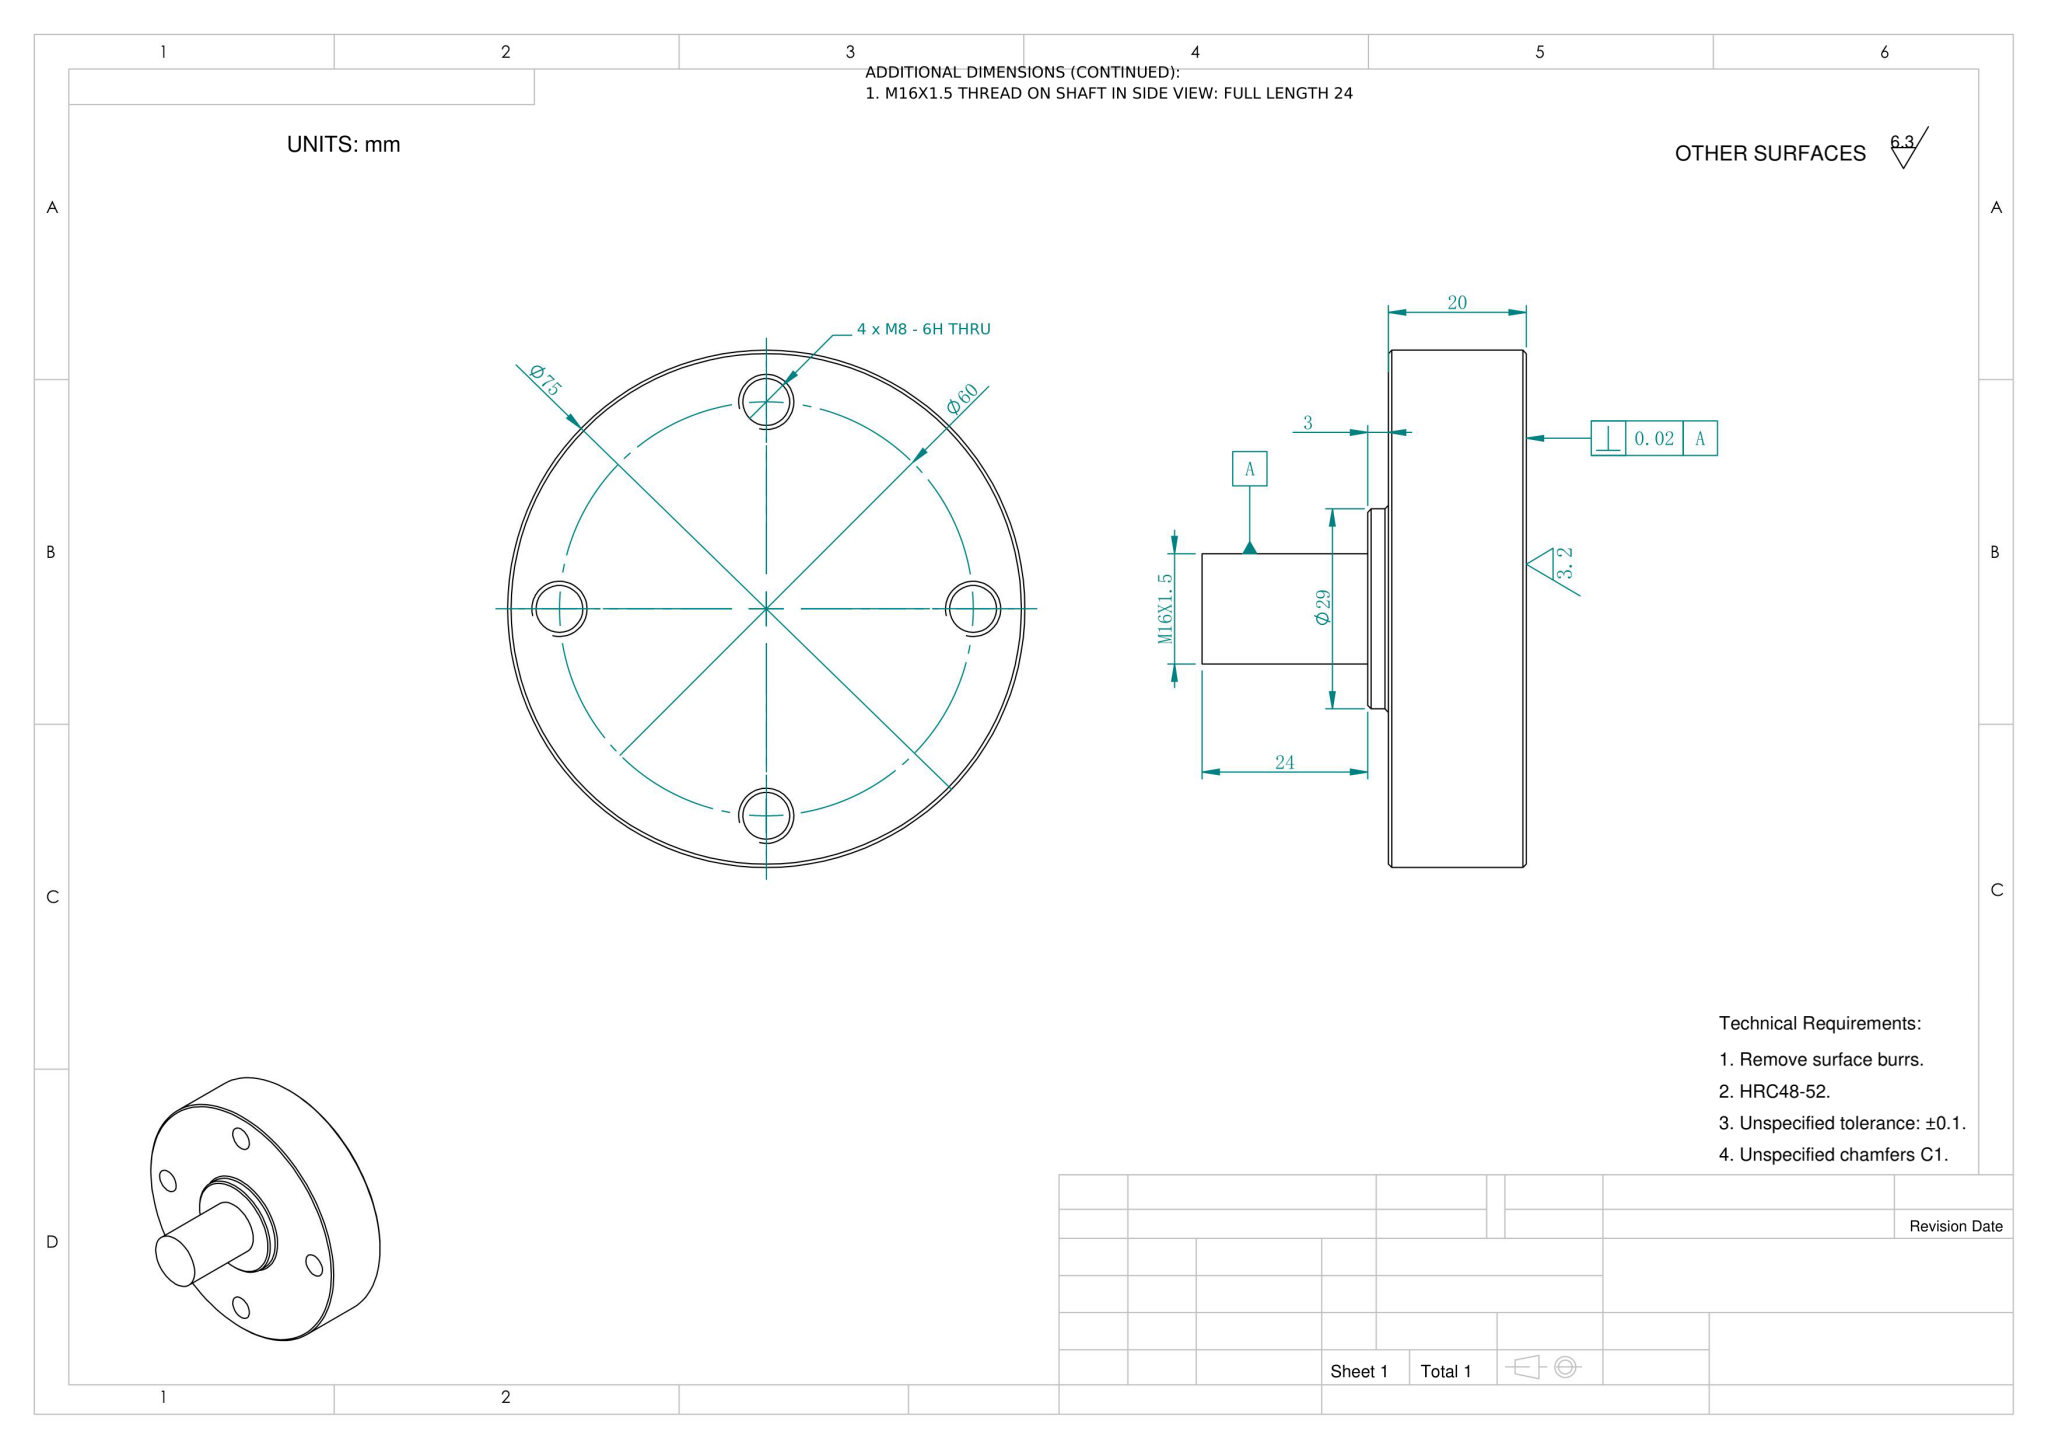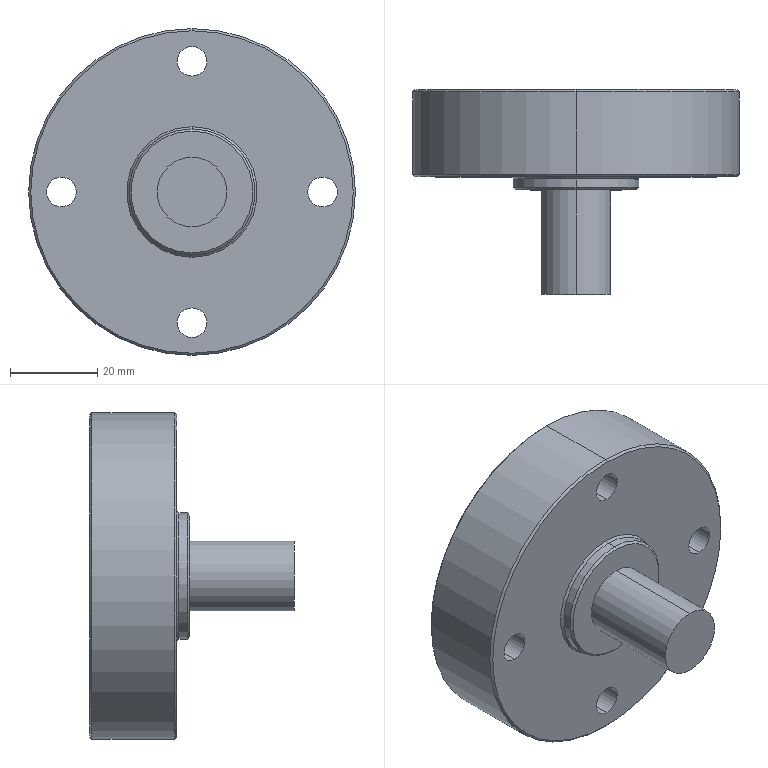Part | NX | mm | 1 solid | 26 faces | box 75 x 47 x 75 mm | volume 92201 mm3 | cylinder 14 | cone 8 | plane 4 | commonest cylinder face diameters 6.8 x8 75 x2 29 x2 16 x2
STEP:
#1=COLOUR_RGB('',0.7922,0.8196,0.9333);
#2=FILL_AREA_STYLE_COLOUR('',#1);
#3=FILL_AREA_STYLE('',(#2));
#4=SURFACE_STYLE_FILL_AREA(#3);
#5=SURFACE_SIDE_STYLE('',(#4));
#6=SURFACE_STYLE_USAGE(.BOTH.,#5);
#7=PRESENTATION_STYLE_ASSIGNMENT((#6));
#8=CARTESIAN_POINT('',(0.,27.,-37.));
#9=VERTEX_POINT('',#8);
#10=CARTESIAN_POINT('',(0.,27.,37.));
#11=VERTEX_POINT('',#10);
#12=CARTESIAN_POINT('',(0.,27.,0.));
#13=DIRECTION('',(0.,-1.,0.));
#14=DIRECTION('',(0.,0.,-1.));
#15=AXIS2_PLACEMENT_3D('',#12,#13,#14);
#16=CIRCLE('',#15,37.);
#17=EDGE_CURVE('',#9,#11,#16,.T.);
#18=ORIENTED_EDGE('',*,*,#17,.F.);
#19=CARTESIAN_POINT('',(0.,27.5,-37.5));
#20=VERTEX_POINT('',#19);
#21=CARTESIAN_POINT('',(0.,27.5,-37.5));
#22=DIRECTION('',(0.,0.7071,-0.7071));
#23=VECTOR('',#22,1000.);
#24=LINE('',#21,#23);
#25=EDGE_CURVE('',#9,#20,#24,.T.);
#26=ORIENTED_EDGE('',*,*,#25,.T.);
#27=CARTESIAN_POINT('',(0.,27.5,37.5));
#28=VERTEX_POINT('',#27);
#29=CARTESIAN_POINT('',(0.,27.5,0.));
#30=DIRECTION('',(0.,1.,0.));
#31=DIRECTION('',(0.,0.,-1.));
#32=AXIS2_PLACEMENT_3D('',#29,#30,#31);
#33=CIRCLE('',#32,37.5);
#34=EDGE_CURVE('',#28,#20,#33,.T.);
#35=ORIENTED_EDGE('',*,*,#34,.F.);
#36=CARTESIAN_POINT('',(0.,27.5,37.5));
#37=DIRECTION('',(0.,0.7071,0.7071));
#38=VECTOR('',#37,1000.);
#39=LINE('',#36,#38);
#40=EDGE_CURVE('',#11,#28,#39,.T.);
#41=ORIENTED_EDGE('',*,*,#40,.F.);
#42=EDGE_LOOP('',(#18,#26,#35,#41));
#43=FACE_OUTER_BOUND('',#42,.T.);
#44=CARTESIAN_POINT('',(0.,27.5,0.));
#45=DIRECTION('',(0.,1.,0.));
#46=DIRECTION('',(0.,0.,1.));
#47=AXIS2_PLACEMENT_3D('',#44,#45,#46);
#48=CONICAL_SURFACE('',#47,37.5,0.7854);
#49=ADVANCED_FACE('',(#43),#48,.T.);
#50=CARTESIAN_POINT('',(0.,47.,37.));
#51=VERTEX_POINT('',#50);
#52=CARTESIAN_POINT('',(0.,47.,-37.));
#53=VERTEX_POINT('',#52);
#54=CARTESIAN_POINT('',(0.,47.,0.));
#55=DIRECTION('',(0.,1.,0.));
#56=DIRECTION('',(0.,0.,1.));
#57=AXIS2_PLACEMENT_3D('',#54,#55,#56);
#58=CIRCLE('',#57,37.);
#59=EDGE_CURVE('',#51,#53,#58,.T.);
#60=ORIENTED_EDGE('',*,*,#59,.F.);
#61=CARTESIAN_POINT('',(0.,46.5,37.5));
#62=VERTEX_POINT('',#61);
#63=CARTESIAN_POINT('',(0.,47.,37.));
#64=DIRECTION('',(0.,-0.7071,0.7071));
#65=VECTOR('',#64,1000.);
#66=LINE('',#63,#65);
#67=EDGE_CURVE('',#51,#62,#66,.T.);
#68=ORIENTED_EDGE('',*,*,#67,.T.);
#69=CARTESIAN_POINT('',(0.,46.5,-37.5));
#70=VERTEX_POINT('',#69);
#71=CARTESIAN_POINT('',(0.,46.5,0.));
#72=DIRECTION('',(0.,-1.,0.));
#73=DIRECTION('',(0.,0.,1.));
#74=AXIS2_PLACEMENT_3D('',#71,#72,#73);
#75=CIRCLE('',#74,37.5);
#76=EDGE_CURVE('',#70,#62,#75,.T.);
#77=ORIENTED_EDGE('',*,*,#76,.F.);
#78=CARTESIAN_POINT('',(0.,47.,-37.));
#79=DIRECTION('',(0.,-0.7071,-0.7071));
#80=VECTOR('',#79,1000.);
#81=LINE('',#78,#80);
#82=EDGE_CURVE('',#53,#70,#81,.T.);
#83=ORIENTED_EDGE('',*,*,#82,.F.);
#84=EDGE_LOOP('',(#60,#68,#77,#83));
#85=FACE_OUTER_BOUND('',#84,.T.);
#86=CARTESIAN_POINT('',(0.,47.,0.));
#87=DIRECTION('',(0.,-1.,0.));
#88=DIRECTION('',(0.,0.,-1.));
#89=AXIS2_PLACEMENT_3D('',#86,#87,#88);
#90=CONICAL_SURFACE('',#89,37.,0.7854);
#91=ADVANCED_FACE('',(#85),#90,.T.);
#92=CARTESIAN_POINT('',(0.,24.,-14.));
#93=VERTEX_POINT('',#92);
#94=CARTESIAN_POINT('',(0.,24.,14.));
#95=VERTEX_POINT('',#94);
#96=CARTESIAN_POINT('',(0.,24.,0.));
#97=DIRECTION('',(0.,-1.,0.));
#98=DIRECTION('',(0.,0.,-1.));
#99=AXIS2_PLACEMENT_3D('',#96,#97,#98);
#100=CIRCLE('',#99,14.);
#101=EDGE_CURVE('',#93,#95,#100,.T.);
#102=ORIENTED_EDGE('',*,*,#101,.F.);
#103=CARTESIAN_POINT('',(0.,24.5,-14.5));
#104=VERTEX_POINT('',#103);
#105=CARTESIAN_POINT('',(0.,24.5,-14.5));
#106=DIRECTION('',(0.,0.7071,-0.7071));
#107=VECTOR('',#106,1000.);
#108=LINE('',#105,#107);
#109=EDGE_CURVE('',#93,#104,#108,.T.);
#110=ORIENTED_EDGE('',*,*,#109,.T.);
#111=CARTESIAN_POINT('',(0.,24.5,14.5));
#112=VERTEX_POINT('',#111);
#113=CARTESIAN_POINT('',(0.,24.5,0.));
#114=DIRECTION('',(0.,1.,0.));
#115=DIRECTION('',(0.,0.,-1.));
#116=AXIS2_PLACEMENT_3D('',#113,#114,#115);
#117=CIRCLE('',#116,14.5);
#118=EDGE_CURVE('',#112,#104,#117,.T.);
#119=ORIENTED_EDGE('',*,*,#118,.F.);
#120=CARTESIAN_POINT('',(0.,24.5,14.5));
#121=DIRECTION('',(0.,0.7071,0.7071));
#122=VECTOR('',#121,1000.);
#123=LINE('',#120,#122);
#124=EDGE_CURVE('',#95,#112,#123,.T.);
#125=ORIENTED_EDGE('',*,*,#124,.F.);
#126=EDGE_LOOP('',(#102,#110,#119,#125));
#127=FACE_OUTER_BOUND('',#126,.T.);
#128=CARTESIAN_POINT('',(0.,24.5,0.));
#129=DIRECTION('',(0.,1.,0.));
#130=DIRECTION('',(0.,0.,1.));
#131=AXIS2_PLACEMENT_3D('',#128,#129,#130);
#132=CONICAL_SURFACE('',#131,14.5,0.7854);
#133=ADVANCED_FACE('',(#127),#132,.T.);
#134=CARTESIAN_POINT('',(0.,26.5,-14.5));
#135=VERTEX_POINT('',#134);
#136=CARTESIAN_POINT('',(0.,26.5,14.5));
#137=VERTEX_POINT('',#136);
#138=CARTESIAN_POINT('',(0.,26.5,0.));
#139=DIRECTION('',(0.,-1.,0.));
#140=DIRECTION('',(0.,0.,-1.));
#141=AXIS2_PLACEMENT_3D('',#138,#139,#140);
#142=CIRCLE('',#141,14.5);
#143=EDGE_CURVE('',#135,#137,#142,.T.);
#144=ORIENTED_EDGE('',*,*,#143,.F.);
#145=CARTESIAN_POINT('',(0.,27.,-15.));
#146=VERTEX_POINT('',#145);
#147=CARTESIAN_POINT('',(0.,27.,-15.));
#148=DIRECTION('',(0.,0.7071,-0.7071));
#149=VECTOR('',#148,1000.);
#150=LINE('',#147,#149);
#151=EDGE_CURVE('',#135,#146,#150,.T.);
#152=ORIENTED_EDGE('',*,*,#151,.T.);
#153=CARTESIAN_POINT('',(0.,27.,15.));
#154=VERTEX_POINT('',#153);
#155=CARTESIAN_POINT('',(0.,27.,0.));
#156=DIRECTION('',(0.,1.,0.));
#157=DIRECTION('',(0.,0.,-1.));
#158=AXIS2_PLACEMENT_3D('',#155,#156,#157);
#159=CIRCLE('',#158,15.);
#160=EDGE_CURVE('',#154,#146,#159,.T.);
#161=ORIENTED_EDGE('',*,*,#160,.F.);
#162=CARTESIAN_POINT('',(0.,27.,15.));
#163=DIRECTION('',(0.,0.7071,0.7071));
#164=VECTOR('',#163,1000.);
#165=LINE('',#162,#164);
#166=EDGE_CURVE('',#137,#154,#165,.T.);
#167=ORIENTED_EDGE('',*,*,#166,.F.);
#168=EDGE_LOOP('',(#144,#152,#161,#167));
#169=FACE_OUTER_BOUND('',#168,.T.);
#170=CARTESIAN_POINT('',(0.,27.,0.));
#171=DIRECTION('',(0.,1.,0.));
#172=DIRECTION('',(0.,0.,1.));
#173=AXIS2_PLACEMENT_3D('',#170,#171,#172);
#174=CONICAL_SURFACE('',#173,15.,0.7854);
#175=ADVANCED_FACE('',(#169),#174,.T.);
#176=CARTESIAN_POINT('',(-30.,27.,3.4));
#177=VERTEX_POINT('',#176);
#178=CARTESIAN_POINT('',(-30.,27.,-3.4));
#179=VERTEX_POINT('',#178);
#180=CARTESIAN_POINT('',(-30.,27.,-0.));
#181=DIRECTION('',(0.,-1.,0.));
#182=DIRECTION('',(0.,0.,-1.));
#183=AXIS2_PLACEMENT_3D('',#180,#181,#182);
#184=CIRCLE('',#183,3.4);
#185=EDGE_CURVE('',#177,#179,#184,.T.);
#186=ORIENTED_EDGE('',*,*,#185,.T.);
#187=CARTESIAN_POINT('',(-30.,47.,-3.4));
#188=VERTEX_POINT('',#187);
#189=CARTESIAN_POINT('',(-30.,47.,-3.4));
#190=DIRECTION('',(0.,1.,0.));
#191=VECTOR('',#190,1000.);
#192=LINE('',#189,#191);
#193=EDGE_CURVE('',#179,#188,#192,.T.);
#194=ORIENTED_EDGE('',*,*,#193,.T.);
#195=CARTESIAN_POINT('',(-30.,47.,3.4));
#196=VERTEX_POINT('',#195);
#197=CARTESIAN_POINT('',(-30.,47.,-0.));
#198=DIRECTION('',(0.,1.,0.));
#199=DIRECTION('',(0.,0.,1.));
#200=AXIS2_PLACEMENT_3D('',#197,#198,#199);
#201=CIRCLE('',#200,3.4);
#202=EDGE_CURVE('',#188,#196,#201,.T.);
#203=ORIENTED_EDGE('',*,*,#202,.T.);
#204=CARTESIAN_POINT('',(-30.,47.,3.4));
#205=DIRECTION('',(0.,1.,0.));
#206=VECTOR('',#205,1000.);
#207=LINE('',#204,#206);
#208=EDGE_CURVE('',#177,#196,#207,.T.);
#209=ORIENTED_EDGE('',*,*,#208,.F.);
#210=EDGE_LOOP('',(#186,#194,#203,#209));
#211=FACE_OUTER_BOUND('',#210,.T.);
#212=CARTESIAN_POINT('',(-30.,47.,-0.));
#213=DIRECTION('',(0.,1.,0.));
#214=DIRECTION('',(0.,0.,1.));
#215=AXIS2_PLACEMENT_3D('',#212,#213,#214);
#216=CYLINDRICAL_SURFACE('',#215,3.4);
#217=ADVANCED_FACE('',(#211),#216,.F.);
#218=CARTESIAN_POINT('',(0.,27.,-26.6));
#219=VERTEX_POINT('',#218);
#220=CARTESIAN_POINT('',(0.,27.,-33.4));
#221=VERTEX_POINT('',#220);
#222=CARTESIAN_POINT('',(0.,27.,-30.));
#223=DIRECTION('',(0.,-1.,0.));
#224=DIRECTION('',(0.,0.,-1.));
#225=AXIS2_PLACEMENT_3D('',#222,#223,#224);
#226=CIRCLE('',#225,3.4);
#227=EDGE_CURVE('',#219,#221,#226,.T.);
#228=ORIENTED_EDGE('',*,*,#227,.T.);
#229=CARTESIAN_POINT('',(0.,47.,-33.4));
#230=VERTEX_POINT('',#229);
#231=CARTESIAN_POINT('',(0.,47.,-33.4));
#232=DIRECTION('',(0.,1.,0.));
#233=VECTOR('',#232,1000.);
#234=LINE('',#231,#233);
#235=EDGE_CURVE('',#221,#230,#234,.T.);
#236=ORIENTED_EDGE('',*,*,#235,.T.);
#237=CARTESIAN_POINT('',(0.,47.,-26.6));
#238=VERTEX_POINT('',#237);
#239=CARTESIAN_POINT('',(0.,47.,-30.));
#240=DIRECTION('',(0.,1.,0.));
#241=DIRECTION('',(0.,0.,1.));
#242=AXIS2_PLACEMENT_3D('',#239,#240,#241);
#243=CIRCLE('',#242,3.4);
#244=EDGE_CURVE('',#230,#238,#243,.T.);
#245=ORIENTED_EDGE('',*,*,#244,.T.);
#246=CARTESIAN_POINT('',(0.,47.,-26.6));
#247=DIRECTION('',(0.,1.,0.));
#248=VECTOR('',#247,1000.);
#249=LINE('',#246,#248);
#250=EDGE_CURVE('',#219,#238,#249,.T.);
#251=ORIENTED_EDGE('',*,*,#250,.F.);
#252=EDGE_LOOP('',(#228,#236,#245,#251));
#253=FACE_OUTER_BOUND('',#252,.T.);
#254=CARTESIAN_POINT('',(0.,47.,-30.));
#255=DIRECTION('',(0.,1.,0.));
#256=DIRECTION('',(0.,0.,1.));
#257=AXIS2_PLACEMENT_3D('',#254,#255,#256);
#258=CYLINDRICAL_SURFACE('',#257,3.4);
#259=ADVANCED_FACE('',(#253),#258,.F.);
#260=CARTESIAN_POINT('',(30.,27.,3.4));
#261=VERTEX_POINT('',#260);
#262=CARTESIAN_POINT('',(30.,27.,-3.4));
#263=VERTEX_POINT('',#262);
#264=CARTESIAN_POINT('',(30.,27.,0.));
#265=DIRECTION('',(0.,-1.,0.));
#266=DIRECTION('',(0.,0.,-1.));
#267=AXIS2_PLACEMENT_3D('',#264,#265,#266);
#268=CIRCLE('',#267,3.4);
#269=EDGE_CURVE('',#261,#263,#268,.T.);
#270=ORIENTED_EDGE('',*,*,#269,.T.);
#271=CARTESIAN_POINT('',(30.,47.,-3.4));
#272=VERTEX_POINT('',#271);
#273=CARTESIAN_POINT('',(30.,47.,-3.4));
#274=DIRECTION('',(0.,1.,0.));
#275=VECTOR('',#274,1000.);
#276=LINE('',#273,#275);
#277=EDGE_CURVE('',#263,#272,#276,.T.);
#278=ORIENTED_EDGE('',*,*,#277,.T.);
#279=CARTESIAN_POINT('',(30.,47.,3.4));
#280=VERTEX_POINT('',#279);
#281=CARTESIAN_POINT('',(30.,47.,0.));
#282=DIRECTION('',(0.,1.,0.));
#283=DIRECTION('',(0.,0.,1.));
#284=AXIS2_PLACEMENT_3D('',#281,#282,#283);
#285=CIRCLE('',#284,3.4);
#286=EDGE_CURVE('',#272,#280,#285,.T.);
#287=ORIENTED_EDGE('',*,*,#286,.T.);
#288=CARTESIAN_POINT('',(30.,47.,3.4));
#289=DIRECTION('',(0.,1.,0.));
#290=VECTOR('',#289,1000.);
#291=LINE('',#288,#290);
#292=EDGE_CURVE('',#261,#280,#291,.T.);
#293=ORIENTED_EDGE('',*,*,#292,.F.);
#294=EDGE_LOOP('',(#270,#278,#287,#293));
#295=FACE_OUTER_BOUND('',#294,.T.);
#296=CARTESIAN_POINT('',(30.,47.,0.));
#297=DIRECTION('',(0.,1.,0.));
#298=DIRECTION('',(0.,0.,1.));
#299=AXIS2_PLACEMENT_3D('',#296,#297,#298);
#300=CYLINDRICAL_SURFACE('',#299,3.4);
#301=ADVANCED_FACE('',(#295),#300,.F.);
#302=CARTESIAN_POINT('',(-0.,27.,33.4));
#303=VERTEX_POINT('',#302);
#304=CARTESIAN_POINT('',(-0.,27.,26.6));
#305=VERTEX_POINT('',#304);
#306=CARTESIAN_POINT('',(-0.,27.,30.));
#307=DIRECTION('',(0.,-1.,0.));
#308=DIRECTION('',(0.,0.,-1.));
#309=AXIS2_PLACEMENT_3D('',#306,#307,#308);
#310=CIRCLE('',#309,3.4);
#311=EDGE_CURVE('',#303,#305,#310,.T.);
#312=ORIENTED_EDGE('',*,*,#311,.T.);
#313=CARTESIAN_POINT('',(-0.,47.,26.6));
#314=VERTEX_POINT('',#313);
#315=CARTESIAN_POINT('',(-0.,47.,26.6));
#316=DIRECTION('',(0.,1.,0.));
#317=VECTOR('',#316,1000.);
#318=LINE('',#315,#317);
#319=EDGE_CURVE('',#305,#314,#318,.T.);
#320=ORIENTED_EDGE('',*,*,#319,.T.);
#321=CARTESIAN_POINT('',(-0.,47.,33.4));
#322=VERTEX_POINT('',#321);
#323=CARTESIAN_POINT('',(-0.,47.,30.));
#324=DIRECTION('',(0.,1.,0.));
#325=DIRECTION('',(0.,0.,1.));
#326=AXIS2_PLACEMENT_3D('',#323,#324,#325);
#327=CIRCLE('',#326,3.4);
#328=EDGE_CURVE('',#314,#322,#327,.T.);
#329=ORIENTED_EDGE('',*,*,#328,.T.);
#330=CARTESIAN_POINT('',(-0.,47.,33.4));
#331=DIRECTION('',(0.,1.,0.));
#332=VECTOR('',#331,1000.);
#333=LINE('',#330,#332);
#334=EDGE_CURVE('',#303,#322,#333,.T.);
#335=ORIENTED_EDGE('',*,*,#334,.F.);
#336=EDGE_LOOP('',(#312,#320,#329,#335));
#337=FACE_OUTER_BOUND('',#336,.T.);
#338=CARTESIAN_POINT('',(-0.,47.,30.));
#339=DIRECTION('',(0.,1.,0.));
#340=DIRECTION('',(0.,0.,1.));
#341=AXIS2_PLACEMENT_3D('',#338,#339,#340);
#342=CYLINDRICAL_SURFACE('',#341,3.4);
#343=ADVANCED_FACE('',(#337),#342,.F.);
#344=ORIENTED_EDGE('',*,*,#34,.T.);
#345=CARTESIAN_POINT('',(0.,47.,-37.5));
#346=DIRECTION('',(0.,1.,0.));
#347=VECTOR('',#346,1000.);
#348=LINE('',#345,#347);
#349=EDGE_CURVE('',#20,#70,#348,.T.);
#350=ORIENTED_EDGE('',*,*,#349,.T.);
#351=ORIENTED_EDGE('',*,*,#76,.T.);
#352=CARTESIAN_POINT('',(0.,47.,37.5));
#353=DIRECTION('',(0.,1.,0.));
#354=VECTOR('',#353,1000.);
#355=LINE('',#352,#354);
#356=EDGE_CURVE('',#28,#62,#355,.T.);
#357=ORIENTED_EDGE('',*,*,#356,.F.);
#358=EDGE_LOOP('',(#344,#350,#351,#357));
#359=FACE_OUTER_BOUND('',#358,.T.);
#360=CARTESIAN_POINT('',(0.,47.,0.));
#361=DIRECTION('',(0.,1.,0.));
#362=DIRECTION('',(0.,0.,1.));
#363=AXIS2_PLACEMENT_3D('',#360,#361,#362);
#364=CYLINDRICAL_SURFACE('',#363,37.5);
#365=ADVANCED_FACE('',(#359),#364,.T.);
#366=ORIENTED_EDGE('',*,*,#118,.T.);
#367=CARTESIAN_POINT('',(0.,47.,-14.5));
#368=DIRECTION('',(0.,1.,0.));
#369=VECTOR('',#368,1000.);
#370=LINE('',#367,#369);
#371=EDGE_CURVE('',#104,#135,#370,.T.);
#372=ORIENTED_EDGE('',*,*,#371,.T.);
#373=ORIENTED_EDGE('',*,*,#143,.T.);
#374=CARTESIAN_POINT('',(0.,47.,14.5));
#375=DIRECTION('',(0.,1.,0.));
#376=VECTOR('',#375,1000.);
#377=LINE('',#374,#376);
#378=EDGE_CURVE('',#112,#137,#377,.T.);
#379=ORIENTED_EDGE('',*,*,#378,.F.);
#380=EDGE_LOOP('',(#366,#372,#373,#379));
#381=FACE_OUTER_BOUND('',#380,.T.);
#382=CARTESIAN_POINT('',(0.,47.,0.));
#383=DIRECTION('',(0.,1.,0.));
#384=DIRECTION('',(0.,0.,1.));
#385=AXIS2_PLACEMENT_3D('',#382,#383,#384);
#386=CYLINDRICAL_SURFACE('',#385,14.5);
#387=ADVANCED_FACE('',(#381),#386,.T.);
#388=CARTESIAN_POINT('',(0.,0.,8.));
#389=VERTEX_POINT('',#388);
#390=CARTESIAN_POINT('',(0.,0.,-8.));
#391=VERTEX_POINT('',#390);
#392=CARTESIAN_POINT('',(0.,0.,0.));
#393=DIRECTION('',(0.,1.,0.));
#394=DIRECTION('',(0.,0.,1.));
#395=AXIS2_PLACEMENT_3D('',#392,#393,#394);
#396=CIRCLE('',#395,8.);
#397=EDGE_CURVE('',#389,#391,#396,.T.);
#398=ORIENTED_EDGE('',*,*,#397,.T.);
#399=CARTESIAN_POINT('',(0.,24.,-8.));
#400=VERTEX_POINT('',#399);
#401=CARTESIAN_POINT('',(0.,47.,-8.));
#402=DIRECTION('',(0.,1.,0.));
#403=VECTOR('',#402,1000.);
#404=LINE('',#401,#403);
#405=EDGE_CURVE('',#391,#400,#404,.T.);
#406=ORIENTED_EDGE('',*,*,#405,.T.);
#407=CARTESIAN_POINT('',(0.,24.,8.));
#408=VERTEX_POINT('',#407);
#409=CARTESIAN_POINT('',(0.,24.,0.));
#410=DIRECTION('',(0.,1.,0.));
#411=DIRECTION('',(0.,0.,1.));
#412=AXIS2_PLACEMENT_3D('',#409,#410,#411);
#413=CIRCLE('',#412,8.);
#414=EDGE_CURVE('',#408,#400,#413,.T.);
#415=ORIENTED_EDGE('',*,*,#414,.F.);
#416=CARTESIAN_POINT('',(0.,47.,8.));
#417=DIRECTION('',(0.,1.,0.));
#418=VECTOR('',#417,1000.);
#419=LINE('',#416,#418);
#420=EDGE_CURVE('',#389,#408,#419,.T.);
#421=ORIENTED_EDGE('',*,*,#420,.F.);
#422=EDGE_LOOP('',(#398,#406,#415,#421));
#423=FACE_OUTER_BOUND('',#422,.T.);
#424=CARTESIAN_POINT('',(0.,47.,0.));
#425=DIRECTION('',(0.,1.,0.));
#426=DIRECTION('',(0.,0.,1.));
#427=AXIS2_PLACEMENT_3D('',#424,#425,#426);
#428=CYLINDRICAL_SURFACE('',#427,8.);
#429=ADVANCED_FACE('',(#423),#428,.T.);
#430=ORIENTED_EDGE('',*,*,#397,.F.);
#431=CARTESIAN_POINT('',(0.,0.,0.));
#432=DIRECTION('',(0.,1.,0.));
#433=DIRECTION('',(0.,0.,1.));
#434=AXIS2_PLACEMENT_3D('',#431,#432,#433);
#435=CIRCLE('',#434,8.);
#436=EDGE_CURVE('',#391,#389,#435,.T.);
#437=ORIENTED_EDGE('',*,*,#436,.F.);
#438=EDGE_LOOP('',(#430,#437));
#439=FACE_OUTER_BOUND('',#438,.T.);
#440=CARTESIAN_POINT('',(0.,0.,0.));
#441=DIRECTION('',(0.,-1.,0.));
#442=DIRECTION('',(0.,0.,-1.));
#443=AXIS2_PLACEMENT_3D('',#440,#441,#442);
#444=PLANE('',#443);
#445=ADVANCED_FACE('',(#439),#444,.T.);
#446=ORIENTED_EDGE('',*,*,#405,.F.);
#447=ORIENTED_EDGE('',*,*,#436,.T.);
#448=ORIENTED_EDGE('',*,*,#420,.T.);
#449=CARTESIAN_POINT('',(0.,24.,0.));
#450=DIRECTION('',(0.,1.,0.));
#451=DIRECTION('',(0.,0.,1.));
#452=AXIS2_PLACEMENT_3D('',#449,#450,#451);
#453=CIRCLE('',#452,8.);
#454=EDGE_CURVE('',#400,#408,#453,.T.);
#455=ORIENTED_EDGE('',*,*,#454,.F.);
#456=EDGE_LOOP('',(#446,#447,#448,#455));
#457=FACE_OUTER_BOUND('',#456,.T.);
#458=CARTESIAN_POINT('',(0.,47.,0.));
#459=DIRECTION('',(0.,1.,0.));
#460=DIRECTION('',(0.,0.,1.));
#461=AXIS2_PLACEMENT_3D('',#458,#459,#460);
#462=CYLINDRICAL_SURFACE('',#461,8.);
#463=ADVANCED_FACE('',(#457),#462,.T.);
#464=CARTESIAN_POINT('',(0.,24.,0.));
#465=DIRECTION('',(0.,-1.,0.));
#466=DIRECTION('',(0.,0.,-1.));
#467=AXIS2_PLACEMENT_3D('',#464,#465,#466);
#468=CIRCLE('',#467,14.);
#469=EDGE_CURVE('',#95,#93,#468,.T.);
#470=ORIENTED_EDGE('',*,*,#469,.T.);
#471=ORIENTED_EDGE('',*,*,#101,.T.);
#472=EDGE_LOOP('',(#470,#471));
#473=FACE_OUTER_BOUND('',#472,.T.);
#474=ORIENTED_EDGE('',*,*,#414,.T.);
#475=ORIENTED_EDGE('',*,*,#454,.T.);
#476=EDGE_LOOP('',(#474,#475));
#477=FACE_BOUND('',#476,.T.);
#478=CARTESIAN_POINT('',(-8.,24.,0.));
#479=DIRECTION('',(0.,-1.,0.));
#480=DIRECTION('',(0.,0.,-1.));
#481=AXIS2_PLACEMENT_3D('',#478,#479,#480);
#482=PLANE('',#481);
#483=ADVANCED_FACE('',(#473,#477),#482,.T.);
#484=ORIENTED_EDGE('',*,*,#371,.F.);
#485=CARTESIAN_POINT('',(0.,24.5,0.));
#486=DIRECTION('',(0.,1.,0.));
#487=DIRECTION('',(0.,0.,-1.));
#488=AXIS2_PLACEMENT_3D('',#485,#486,#487);
#489=CIRCLE('',#488,14.5);
#490=EDGE_CURVE('',#104,#112,#489,.T.);
#491=ORIENTED_EDGE('',*,*,#490,.T.);
#492=ORIENTED_EDGE('',*,*,#378,.T.);
#493=CARTESIAN_POINT('',(0.,26.5,0.));
#494=DIRECTION('',(0.,-1.,0.));
#495=DIRECTION('',(0.,0.,-1.));
#496=AXIS2_PLACEMENT_3D('',#493,#494,#495);
#497=CIRCLE('',#496,14.5);
#498=EDGE_CURVE('',#137,#135,#497,.T.);
#499=ORIENTED_EDGE('',*,*,#498,.T.);
#500=EDGE_LOOP('',(#484,#491,#492,#499));
#501=FACE_OUTER_BOUND('',#500,.T.);
#502=CARTESIAN_POINT('',(0.,47.,0.));
#503=DIRECTION('',(0.,1.,0.));
#504=DIRECTION('',(0.,0.,1.));
#505=AXIS2_PLACEMENT_3D('',#502,#503,#504);
#506=CYLINDRICAL_SURFACE('',#505,14.5);
#507=ADVANCED_FACE('',(#501),#506,.T.);
#508=ORIENTED_EDGE('',*,*,#160,.T.);
#509=CARTESIAN_POINT('',(0.,27.,0.));
#510=DIRECTION('',(0.,1.,0.));
#511=DIRECTION('',(0.,0.,-1.));
#512=AXIS2_PLACEMENT_3D('',#509,#510,#511);
#513=CIRCLE('',#512,15.);
#514=EDGE_CURVE('',#146,#154,#513,.T.);
#515=ORIENTED_EDGE('',*,*,#514,.T.);
#516=EDGE_LOOP('',(#508,#515));
#517=FACE_BOUND('',#516,.T.);
#518=CARTESIAN_POINT('',(0.,27.,0.));
#519=DIRECTION('',(0.,-1.,0.));
#520=DIRECTION('',(0.,0.,-1.));
#521=AXIS2_PLACEMENT_3D('',#518,#519,#520);
#522=CIRCLE('',#521,37.);
#523=EDGE_CURVE('',#11,#9,#522,.T.);
#524=ORIENTED_EDGE('',*,*,#523,.T.);
#525=ORIENTED_EDGE('',*,*,#17,.T.);
#526=EDGE_LOOP('',(#524,#525));
#527=FACE_OUTER_BOUND('',#526,.T.);
#528=ORIENTED_EDGE('',*,*,#185,.F.);
#529=CARTESIAN_POINT('',(-30.,27.,-0.));
#530=DIRECTION('',(0.,-1.,0.));
#531=DIRECTION('',(0.,0.,-1.));
#532=AXIS2_PLACEMENT_3D('',#529,#530,#531);
#533=CIRCLE('',#532,3.4);
#534=EDGE_CURVE('',#179,#177,#533,.T.);
#535=ORIENTED_EDGE('',*,*,#534,.F.);
#536=EDGE_LOOP('',(#528,#535));
#537=FACE_BOUND('',#536,.T.);
#538=ORIENTED_EDGE('',*,*,#227,.F.);
#539=CARTESIAN_POINT('',(0.,27.,-30.));
#540=DIRECTION('',(0.,-1.,0.));
#541=DIRECTION('',(0.,0.,-1.));
#542=AXIS2_PLACEMENT_3D('',#539,#540,#541);
#543=CIRCLE('',#542,3.4);
#544=EDGE_CURVE('',#221,#219,#543,.T.);
#545=ORIENTED_EDGE('',*,*,#544,.F.);
#546=EDGE_LOOP('',(#538,#545));
#547=FACE_BOUND('',#546,.T.);
#548=ORIENTED_EDGE('',*,*,#269,.F.);
#549=CARTESIAN_POINT('',(30.,27.,0.));
#550=DIRECTION('',(0.,-1.,0.));
#551=DIRECTION('',(0.,0.,-1.));
#552=AXIS2_PLACEMENT_3D('',#549,#550,#551);
#553=CIRCLE('',#552,3.4);
#554=EDGE_CURVE('',#263,#261,#553,.T.);
#555=ORIENTED_EDGE('',*,*,#554,.F.);
#556=EDGE_LOOP('',(#548,#555));
#557=FACE_BOUND('',#556,.T.);
#558=ORIENTED_EDGE('',*,*,#311,.F.);
#559=CARTESIAN_POINT('',(-0.,27.,30.));
#560=DIRECTION('',(0.,-1.,0.));
#561=DIRECTION('',(0.,0.,-1.));
#562=AXIS2_PLACEMENT_3D('',#559,#560,#561);
#563=CIRCLE('',#562,3.4);
#564=EDGE_CURVE('',#305,#303,#563,.T.);
#565=ORIENTED_EDGE('',*,*,#564,.F.);
#566=EDGE_LOOP('',(#558,#565));
#567=FACE_BOUND('',#566,.T.);
#568=CARTESIAN_POINT('',(-14.5,27.,0.));
#569=DIRECTION('',(0.,-1.,0.));
#570=DIRECTION('',(0.,0.,-1.));
#571=AXIS2_PLACEMENT_3D('',#568,#569,#570);
#572=PLANE('',#571);
#573=ADVANCED_FACE('',(#517,#527,#537,#547,#557,#567),#572,.T.);
#574=ORIENTED_EDGE('',*,*,#349,.F.);
#575=CARTESIAN_POINT('',(0.,27.5,0.));
#576=DIRECTION('',(0.,1.,0.));
#577=DIRECTION('',(0.,0.,-1.));
#578=AXIS2_PLACEMENT_3D('',#575,#576,#577);
#579=CIRCLE('',#578,37.5);
#580=EDGE_CURVE('',#20,#28,#579,.T.);
#581=ORIENTED_EDGE('',*,*,#580,.T.);
#582=ORIENTED_EDGE('',*,*,#356,.T.);
#583=CARTESIAN_POINT('',(0.,46.5,0.));
#584=DIRECTION('',(0.,-1.,0.));
#585=DIRECTION('',(0.,0.,1.));
#586=AXIS2_PLACEMENT_3D('',#583,#584,#585);
#587=CIRCLE('',#586,37.5);
#588=EDGE_CURVE('',#62,#70,#587,.T.);
#589=ORIENTED_EDGE('',*,*,#588,.T.);
#590=EDGE_LOOP('',(#574,#581,#582,#589));
#591=FACE_OUTER_BOUND('',#590,.T.);
#592=CARTESIAN_POINT('',(0.,47.,0.));
#593=DIRECTION('',(0.,1.,0.));
#594=DIRECTION('',(0.,0.,1.));
#595=AXIS2_PLACEMENT_3D('',#592,#593,#594);
#596=CYLINDRICAL_SURFACE('',#595,37.5);
#597=ADVANCED_FACE('',(#591),#596,.T.);
#598=CARTESIAN_POINT('',(0.,47.,0.));
#599=DIRECTION('',(0.,1.,0.));
#600=DIRECTION('',(0.,0.,1.));
#601=AXIS2_PLACEMENT_3D('',#598,#599,#600);
#602=CIRCLE('',#601,37.);
#603=EDGE_CURVE('',#53,#51,#602,.T.);
#604=ORIENTED_EDGE('',*,*,#603,.T.);
#605=ORIENTED_EDGE('',*,*,#59,.T.);
#606=EDGE_LOOP('',(#604,#605));
#607=FACE_OUTER_BOUND('',#606,.T.);
#608=CARTESIAN_POINT('',(-30.,47.,-0.));
#609=DIRECTION('',(0.,1.,0.));
#610=DIRECTION('',(0.,0.,1.));
#611=AXIS2_PLACEMENT_3D('',#608,#609,#610);
#612=CIRCLE('',#611,3.4);
#613=EDGE_CURVE('',#196,#188,#612,.T.);
#614=ORIENTED_EDGE('',*,*,#613,.F.);
#615=ORIENTED_EDGE('',*,*,#202,.F.);
#616=EDGE_LOOP('',(#614,#615));
#617=FACE_BOUND('',#616,.T.);
#618=CARTESIAN_POINT('',(0.,47.,-30.));
#619=DIRECTION('',(0.,1.,0.));
#620=DIRECTION('',(0.,0.,1.));
#621=AXIS2_PLACEMENT_3D('',#618,#619,#620);
#622=CIRCLE('',#621,3.4);
#623=EDGE_CURVE('',#238,#230,#622,.T.);
#624=ORIENTED_EDGE('',*,*,#623,.F.);
#625=ORIENTED_EDGE('',*,*,#244,.F.);
#626=EDGE_LOOP('',(#624,#625));
#627=FACE_BOUND('',#626,.T.);
#628=CARTESIAN_POINT('',(30.,47.,0.));
#629=DIRECTION('',(0.,1.,0.));
#630=DIRECTION('',(0.,0.,1.));
#631=AXIS2_PLACEMENT_3D('',#628,#629,#630);
#632=CIRCLE('',#631,3.4);
#633=EDGE_CURVE('',#280,#272,#632,.T.);
#634=ORIENTED_EDGE('',*,*,#633,.F.);
#635=ORIENTED_EDGE('',*,*,#286,.F.);
#636=EDGE_LOOP('',(#634,#635));
#637=FACE_BOUND('',#636,.T.);
#638=CARTESIAN_POINT('',(-0.,47.,30.));
#639=DIRECTION('',(0.,1.,0.));
#640=DIRECTION('',(0.,0.,1.));
#641=AXIS2_PLACEMENT_3D('',#638,#639,#640);
#642=CIRCLE('',#641,3.4);
#643=EDGE_CURVE('',#322,#314,#642,.T.);
#644=ORIENTED_EDGE('',*,*,#643,.F.);
#645=ORIENTED_EDGE('',*,*,#328,.F.);
#646=EDGE_LOOP('',(#644,#645));
#647=FACE_BOUND('',#646,.T.);
#648=CARTESIAN_POINT('',(-37.5,47.,0.));
#649=DIRECTION('',(0.,1.,0.));
#650=DIRECTION('',(0.,0.,1.));
#651=AXIS2_PLACEMENT_3D('',#648,#649,#650);
#652=PLANE('',#651);
#653=ADVANCED_FACE('',(#607,#617,#627,#637,#647),#652,.T.);
#654=ORIENTED_EDGE('',*,*,#319,.F.);
#655=ORIENTED_EDGE('',*,*,#564,.T.);
#656=ORIENTED_EDGE('',*,*,#334,.T.);
#657=ORIENTED_EDGE('',*,*,#643,.T.);
#658=EDGE_LOOP('',(#654,#655,#656,#657));
#659=FACE_OUTER_BOUND('',#658,.T.);
#660=CARTESIAN_POINT('',(-0.,47.,30.));
#661=DIRECTION('',(0.,1.,0.));
#662=DIRECTION('',(0.,0.,1.));
#663=AXIS2_PLACEMENT_3D('',#660,#661,#662);
#664=CYLINDRICAL_SURFACE('',#663,3.4);
#665=ADVANCED_FACE('',(#659),#664,.F.);
#666=ORIENTED_EDGE('',*,*,#277,.F.);
#667=ORIENTED_EDGE('',*,*,#554,.T.);
#668=ORIENTED_EDGE('',*,*,#292,.T.);
#669=ORIENTED_EDGE('',*,*,#633,.T.);
#670=EDGE_LOOP('',(#666,#667,#668,#669));
#671=FACE_OUTER_BOUND('',#670,.T.);
#672=CARTESIAN_POINT('',(30.,47.,0.));
#673=DIRECTION('',(0.,1.,0.));
#674=DIRECTION('',(0.,0.,1.));
#675=AXIS2_PLACEMENT_3D('',#672,#673,#674);
#676=CYLINDRICAL_SURFACE('',#675,3.4);
#677=ADVANCED_FACE('',(#671),#676,.F.);
#678=ORIENTED_EDGE('',*,*,#235,.F.);
#679=ORIENTED_EDGE('',*,*,#544,.T.);
#680=ORIENTED_EDGE('',*,*,#250,.T.);
#681=ORIENTED_EDGE('',*,*,#623,.T.);
#682=EDGE_LOOP('',(#678,#679,#680,#681));
#683=FACE_OUTER_BOUND('',#682,.T.);
#684=CARTESIAN_POINT('',(0.,47.,-30.));
#685=DIRECTION('',(0.,1.,0.));
#686=DIRECTION('',(0.,0.,1.));
#687=AXIS2_PLACEMENT_3D('',#684,#685,#686);
#688=CYLINDRICAL_SURFACE('',#687,3.4);
#689=ADVANCED_FACE('',(#683),#688,.F.);
#690=ORIENTED_EDGE('',*,*,#193,.F.);
#691=ORIENTED_EDGE('',*,*,#534,.T.);
#692=ORIENTED_EDGE('',*,*,#208,.T.);
#693=ORIENTED_EDGE('',*,*,#613,.T.);
#694=EDGE_LOOP('',(#690,#691,#692,#693));
#695=FACE_OUTER_BOUND('',#694,.T.);
#696=CARTESIAN_POINT('',(-30.,47.,-0.));
#697=DIRECTION('',(0.,1.,0.));
#698=DIRECTION('',(0.,0.,1.));
#699=AXIS2_PLACEMENT_3D('',#696,#697,#698);
#700=CYLINDRICAL_SURFACE('',#699,3.4);
#701=ADVANCED_FACE('',(#695),#700,.F.);
#702=ORIENTED_EDGE('',*,*,#151,.F.);
#703=ORIENTED_EDGE('',*,*,#498,.F.);
#704=ORIENTED_EDGE('',*,*,#166,.T.);
#705=ORIENTED_EDGE('',*,*,#514,.F.);
#706=EDGE_LOOP('',(#702,#703,#704,#705));
#707=FACE_OUTER_BOUND('',#706,.T.);
#708=CARTESIAN_POINT('',(0.,27.,0.));
#709=DIRECTION('',(0.,1.,0.));
#710=DIRECTION('',(0.,0.,1.));
#711=AXIS2_PLACEMENT_3D('',#708,#709,#710);
#712=CONICAL_SURFACE('',#711,15.,0.7854);
#713=ADVANCED_FACE('',(#707),#712,.T.);
#714=ORIENTED_EDGE('',*,*,#109,.F.);
#715=ORIENTED_EDGE('',*,*,#469,.F.);
#716=ORIENTED_EDGE('',*,*,#124,.T.);
#717=ORIENTED_EDGE('',*,*,#490,.F.);
#718=EDGE_LOOP('',(#714,#715,#716,#717));
#719=FACE_OUTER_BOUND('',#718,.T.);
#720=CARTESIAN_POINT('',(0.,24.5,0.));
#721=DIRECTION('',(0.,1.,0.));
#722=DIRECTION('',(0.,0.,1.));
#723=AXIS2_PLACEMENT_3D('',#720,#721,#722);
#724=CONICAL_SURFACE('',#723,14.5,0.7854);
#725=ADVANCED_FACE('',(#719),#724,.T.);
#726=ORIENTED_EDGE('',*,*,#67,.F.);
#727=ORIENTED_EDGE('',*,*,#603,.F.);
#728=ORIENTED_EDGE('',*,*,#82,.T.);
#729=ORIENTED_EDGE('',*,*,#588,.F.);
#730=EDGE_LOOP('',(#726,#727,#728,#729));
#731=FACE_OUTER_BOUND('',#730,.T.);
#732=CARTESIAN_POINT('',(0.,47.,0.));
#733=DIRECTION('',(0.,-1.,0.));
#734=DIRECTION('',(0.,0.,-1.));
#735=AXIS2_PLACEMENT_3D('',#732,#733,#734);
#736=CONICAL_SURFACE('',#735,37.,0.7854);
#737=ADVANCED_FACE('',(#731),#736,.T.);
#738=ORIENTED_EDGE('',*,*,#25,.F.);
#739=ORIENTED_EDGE('',*,*,#523,.F.);
#740=ORIENTED_EDGE('',*,*,#40,.T.);
#741=ORIENTED_EDGE('',*,*,#580,.F.);
#742=EDGE_LOOP('',(#738,#739,#740,#741));
#743=FACE_OUTER_BOUND('',#742,.T.);
#744=CARTESIAN_POINT('',(0.,27.5,0.));
#745=DIRECTION('',(0.,1.,0.));
#746=DIRECTION('',(0.,0.,1.));
#747=AXIS2_PLACEMENT_3D('',#744,#745,#746);
#748=CONICAL_SURFACE('',#747,37.5,0.7854);
#749=ADVANCED_FACE('',(#743),#748,.T.);
#750=CLOSED_SHELL('',(#49,#91,#133,#175,#217,#259,#301,#343,#365,#387,#429,#445,#463,#483,#507,#573,#597,#653,#665,#677,#689,#701,#713,#725,#737,#749));
#751=MANIFOLD_SOLID_BREP('',#750);
#752=STYLED_ITEM('',(#7),#751);
#753=PRESENTATION_LAYER_ASSIGNMENT('','',(#752));
#754=CARTESIAN_POINT('',(0.,0.,0.));
#755=DIRECTION('',(0.,0.,1.));
#756=DIRECTION('',(1.,0.,0.));
#757=AXIS2_PLACEMENT_3D('',#754,#755,#756);
#758=(LENGTH_UNIT()NAMED_UNIT(*)SI_UNIT(.MILLI.,.METRE.));
#759=UNCERTAINTY_MEASURE_WITH_UNIT(LENGTH_MEASURE(0.00001),#758,'','');
#760=(NAMED_UNIT(*)PLANE_ANGLE_UNIT()SI_UNIT($,.RADIAN.));
#761=(NAMED_UNIT(*)SI_UNIT($,.STERADIAN.)SOLID_ANGLE_UNIT());
#762=(GEOMETRIC_REPRESENTATION_CONTEXT(3)GLOBAL_UNCERTAINTY_ASSIGNED_CONTEXT((#759))GLOBAL_UNIT_ASSIGNED_CONTEXT((#758,#760,#761))REPRESENTATION_CONTEXT('',''));
#763=ADVANCED_BREP_SHAPE_REPRESENTATION('',(#751,#757),#762);
#764=(LENGTH_UNIT()NAMED_UNIT(*)SI_UNIT(.MILLI.,.METRE.));
#765=UNCERTAINTY_MEASURE_WITH_UNIT(LENGTH_MEASURE(0.00001),#764,'','');
#766=(NAMED_UNIT(*)PLANE_ANGLE_UNIT()SI_UNIT($,.RADIAN.));
#767=(NAMED_UNIT(*)SI_UNIT($,.STERADIAN.)SOLID_ANGLE_UNIT());
#768=(GEOMETRIC_REPRESENTATION_CONTEXT(3)GLOBAL_UNCERTAINTY_ASSIGNED_CONTEXT((#765))GLOBAL_UNIT_ASSIGNED_CONTEXT((#764,#766,#767))REPRESENTATION_CONTEXT('',''));
#769=MECHANICAL_DESIGN_GEOMETRIC_PRESENTATION_REPRESENTATION('',(#752),#768);